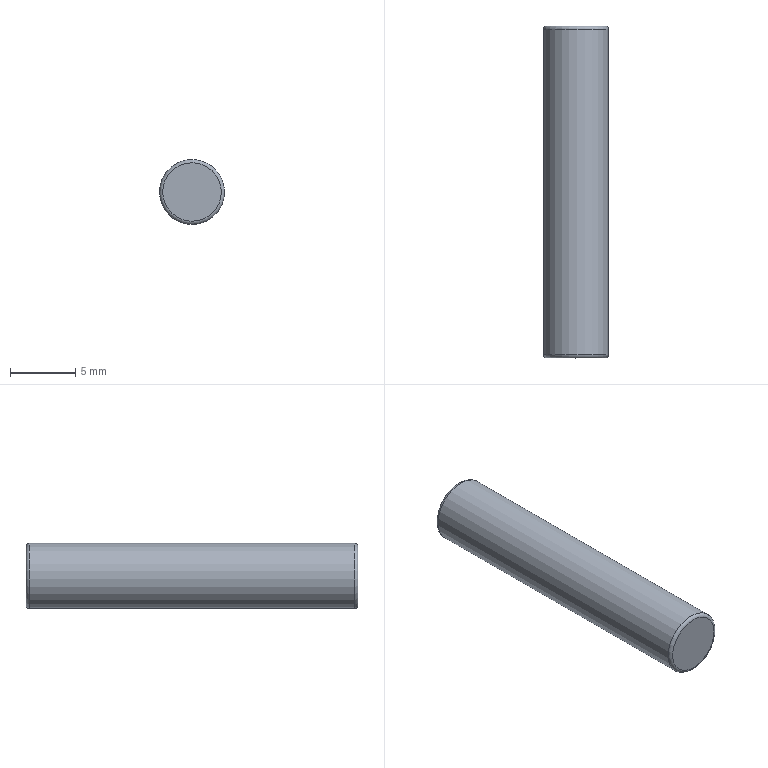Component | NX | PISTON_PIN | 1 solid | 5 faces | volume 500 mm3 | plane 2 | torus 2 | cylinder 1 | commonest cylinder face diameters 5 x1